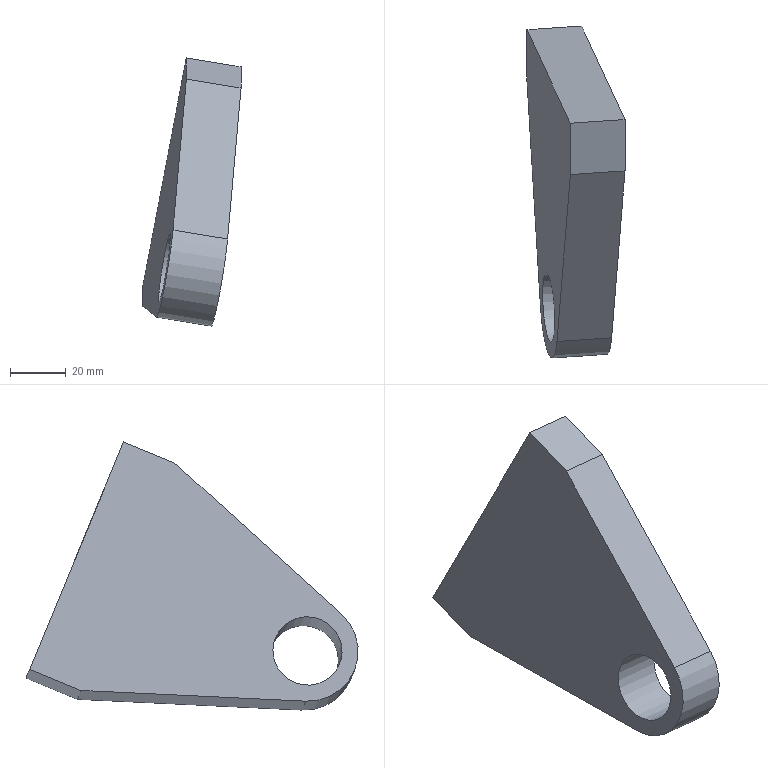Component | NX | 4 | 1 solid | 9 faces | volume 127186 mm3 | plane 7 | cylinder 2 | commonest cylinder face diameters 36.69 x1 25 x1